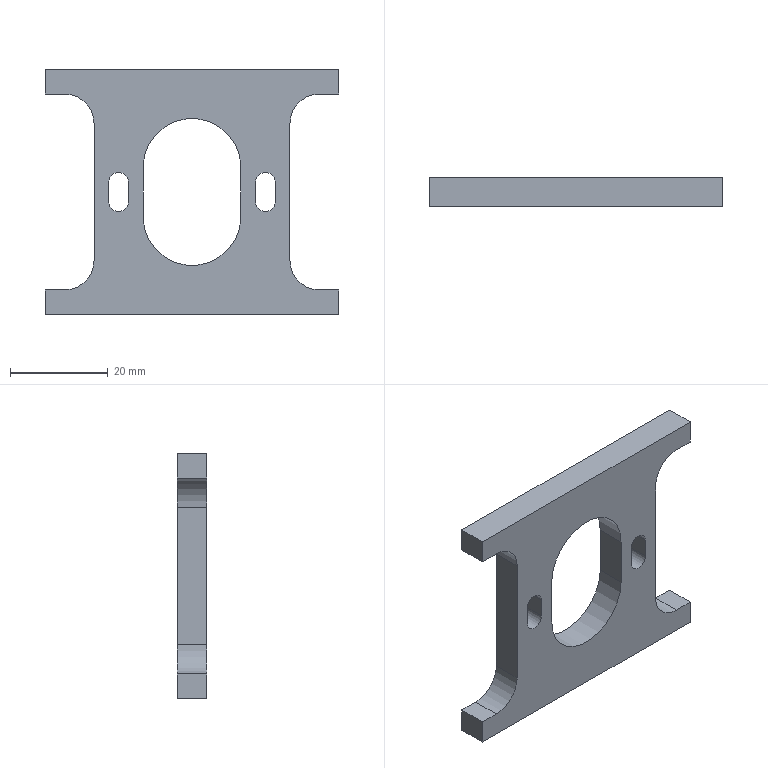Component | NX | SLIDE_PLATE_2 | 1 solid | 30 faces | volume 9958 mm3 | plane 20 | cylinder 10 | commonest cylinder face diameters 12 x4 4 x4 20 x2